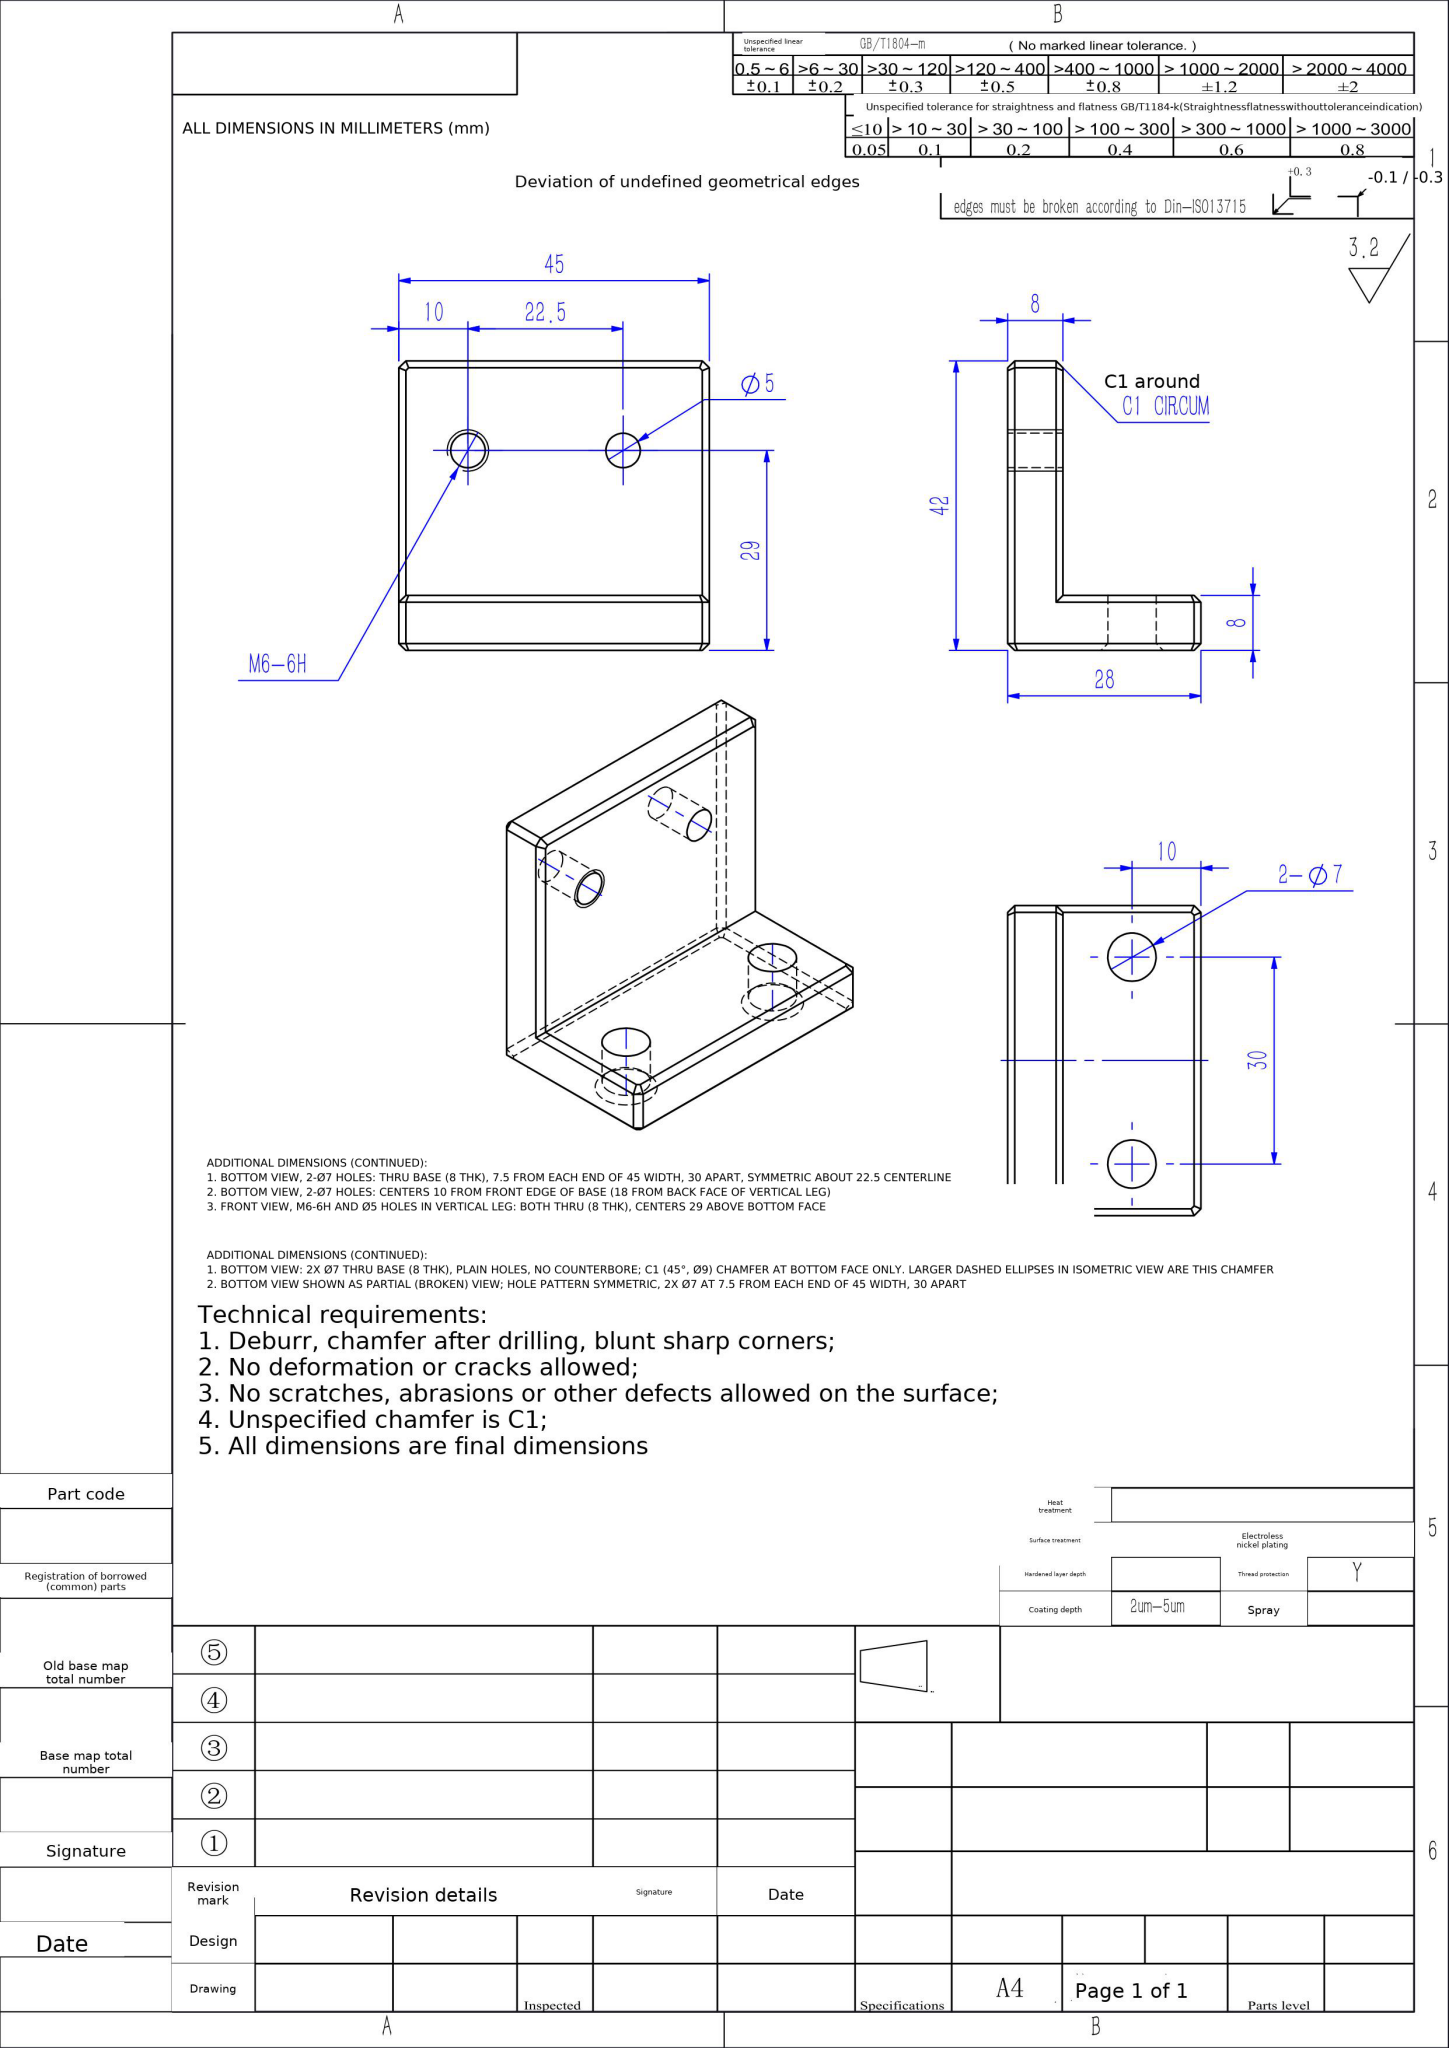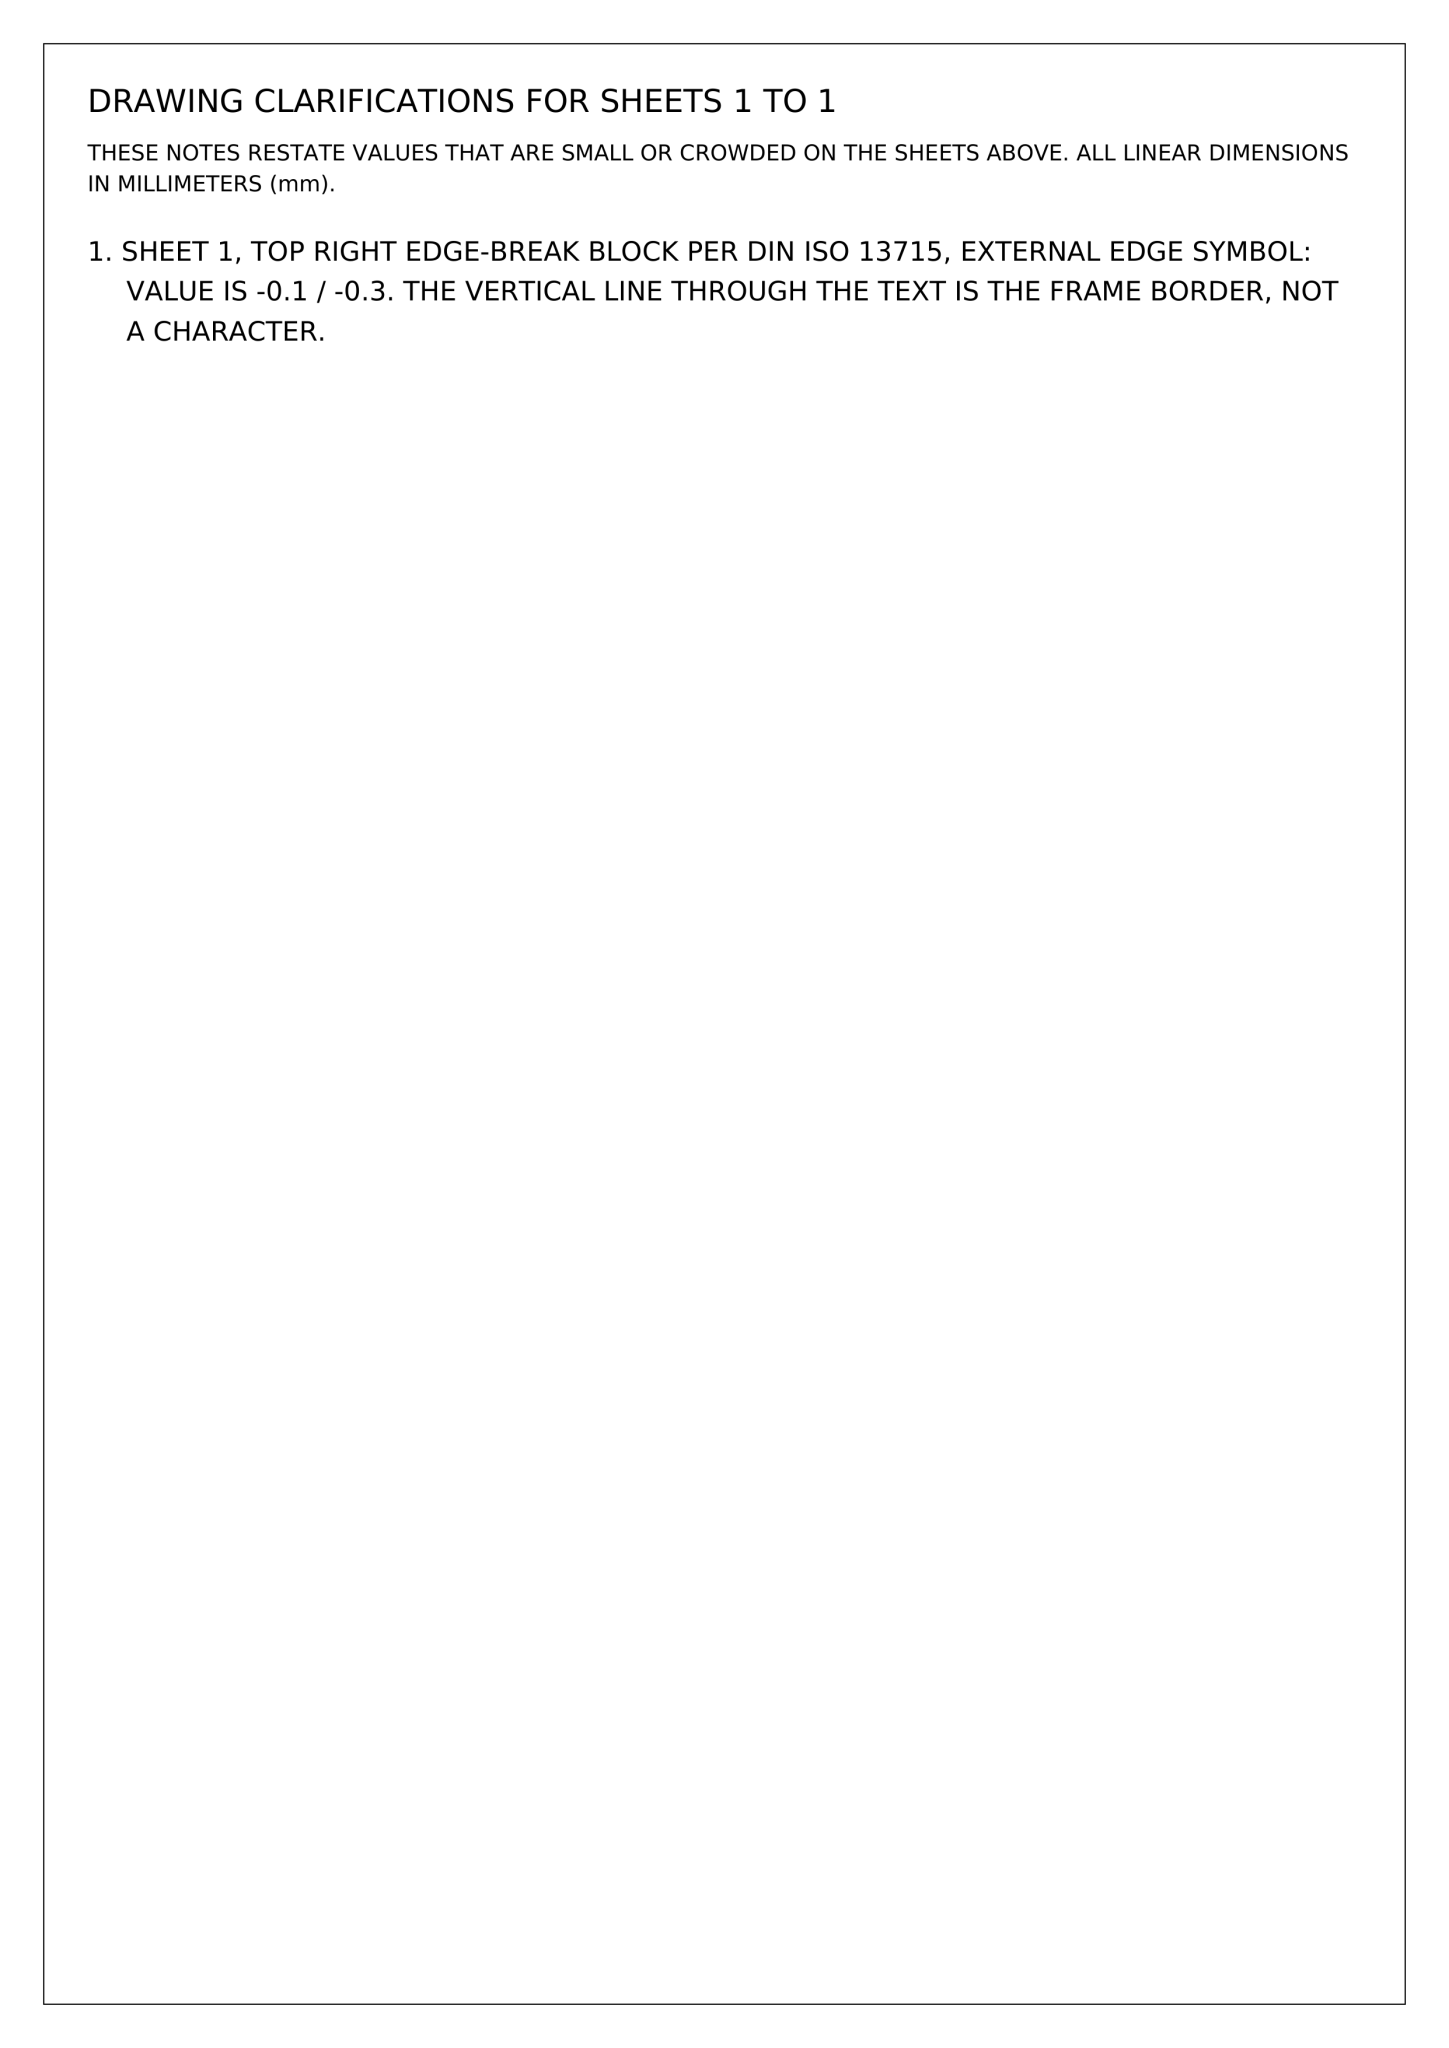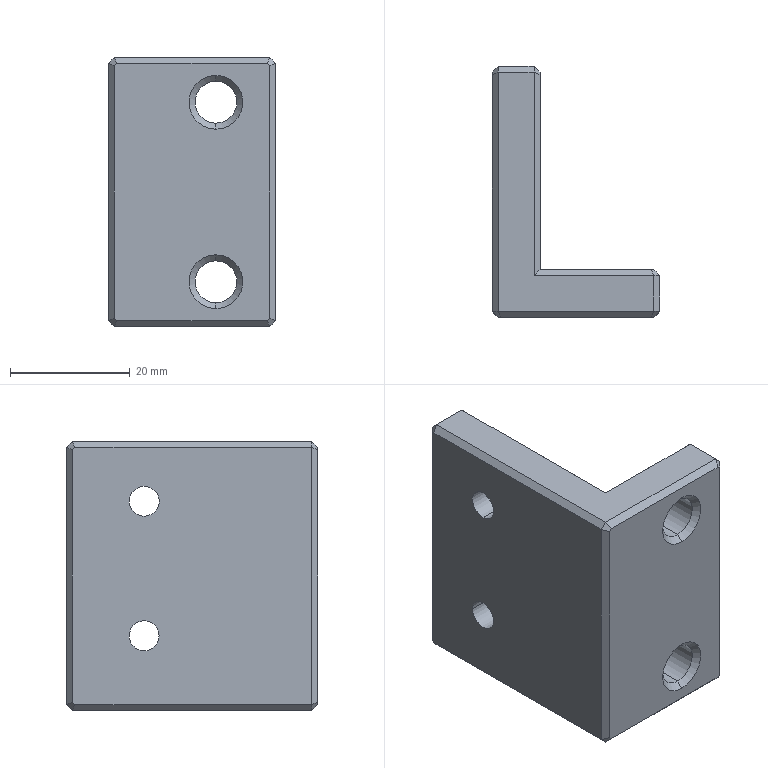Part | NX | mm | 1 solid | 47 faces | box 28 x 42 x 45 mm | volume 21119 mm3 | plane 35 | cylinder 8 | cone 4 | commonest cylinder face diameters 5 x4 7 x4